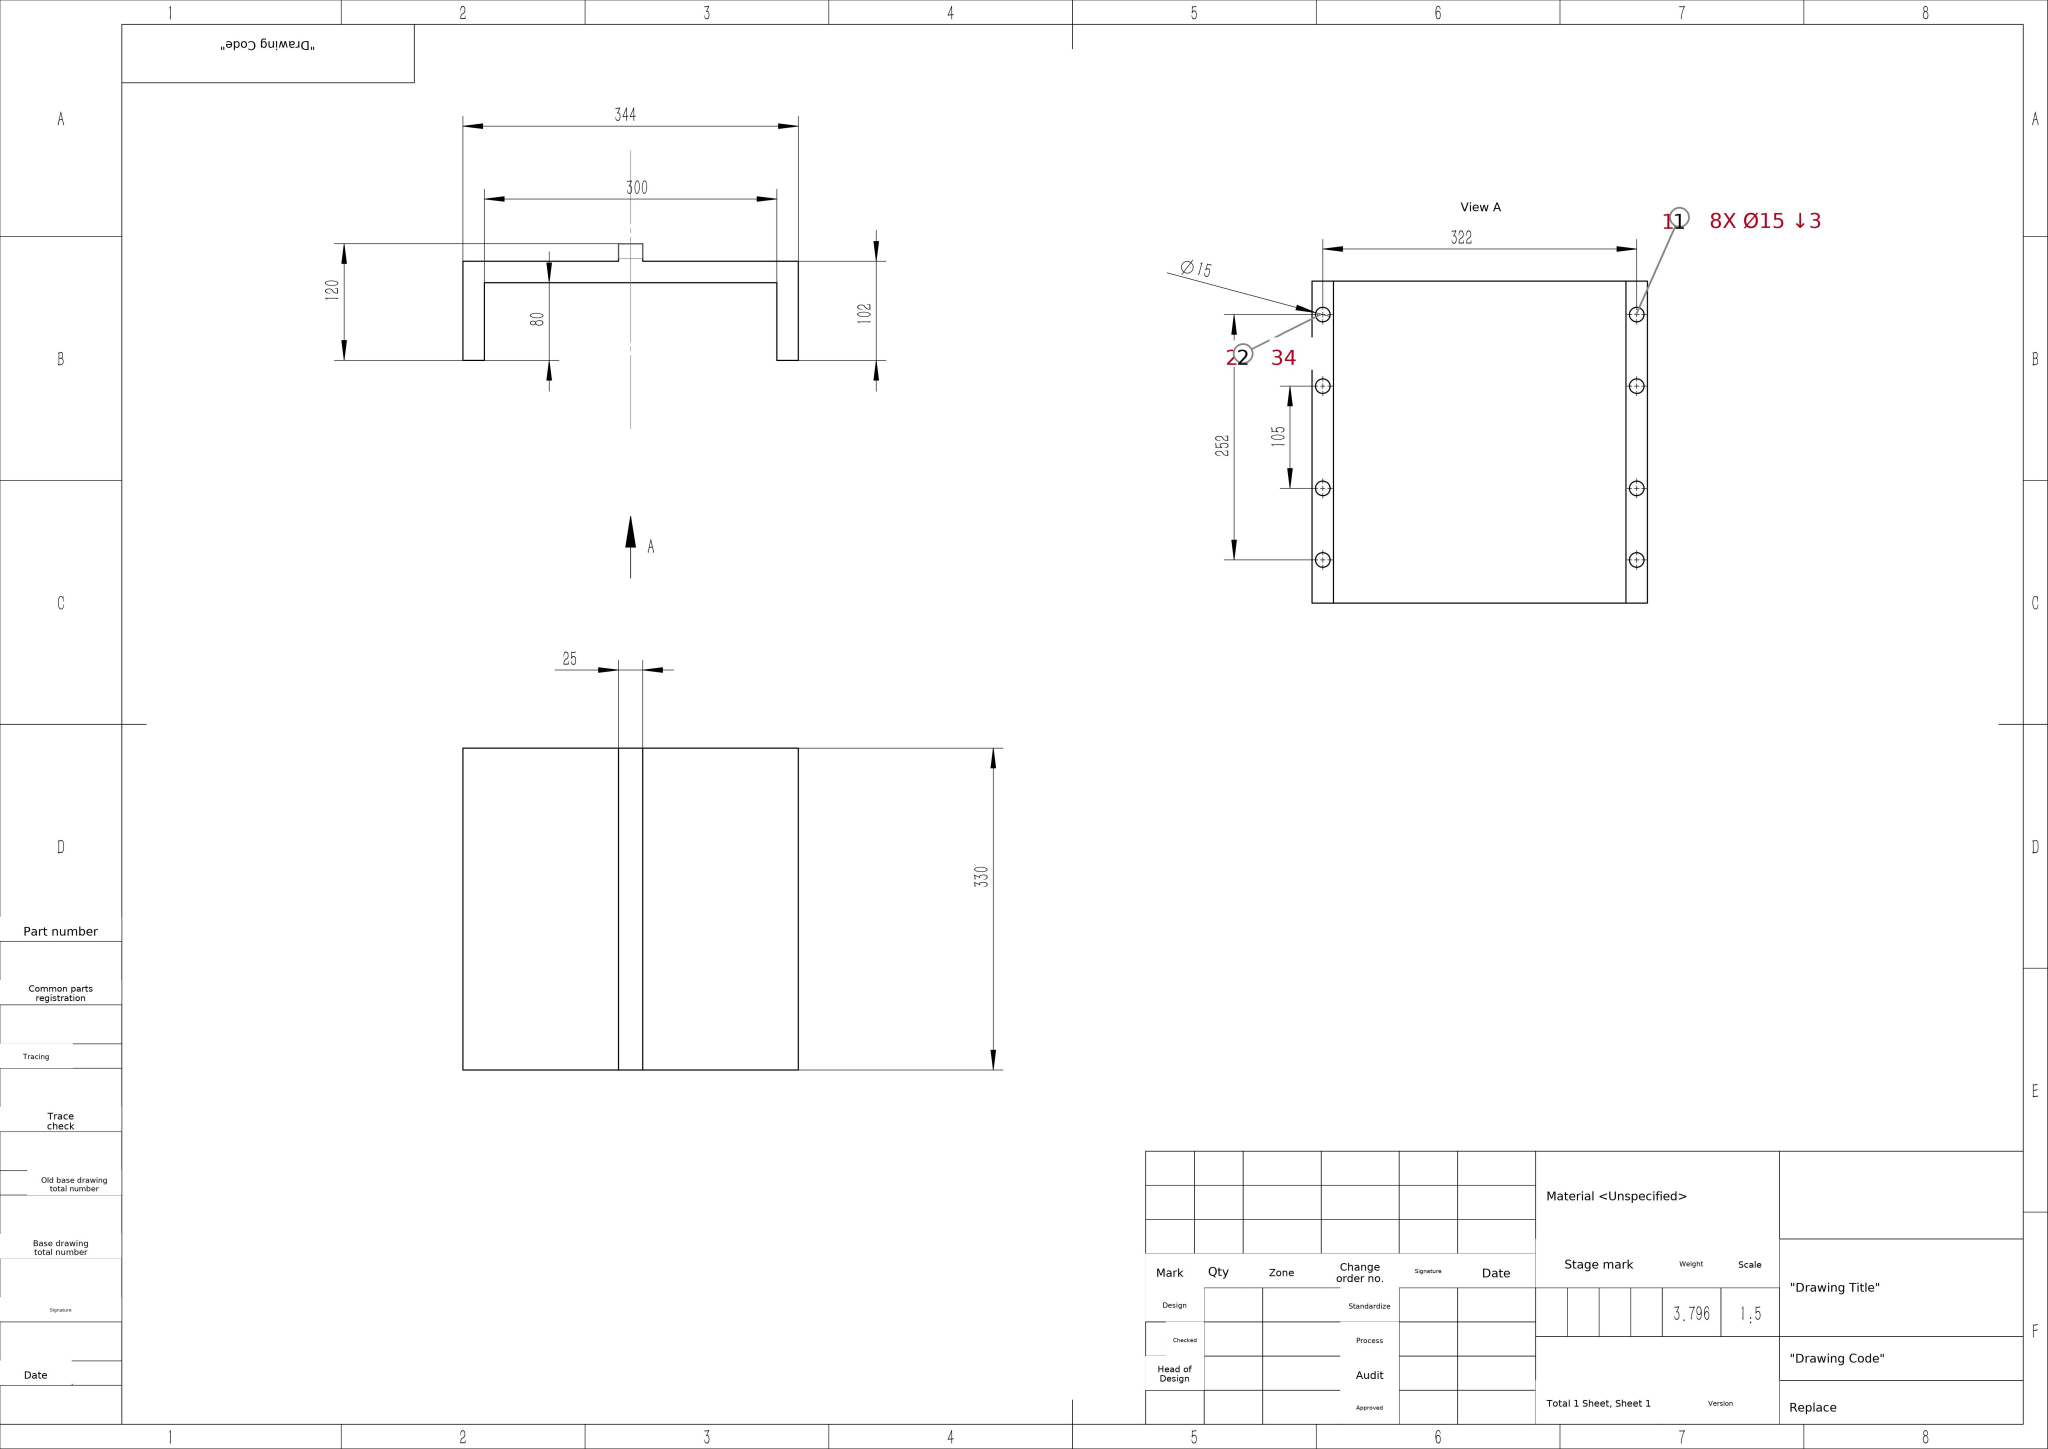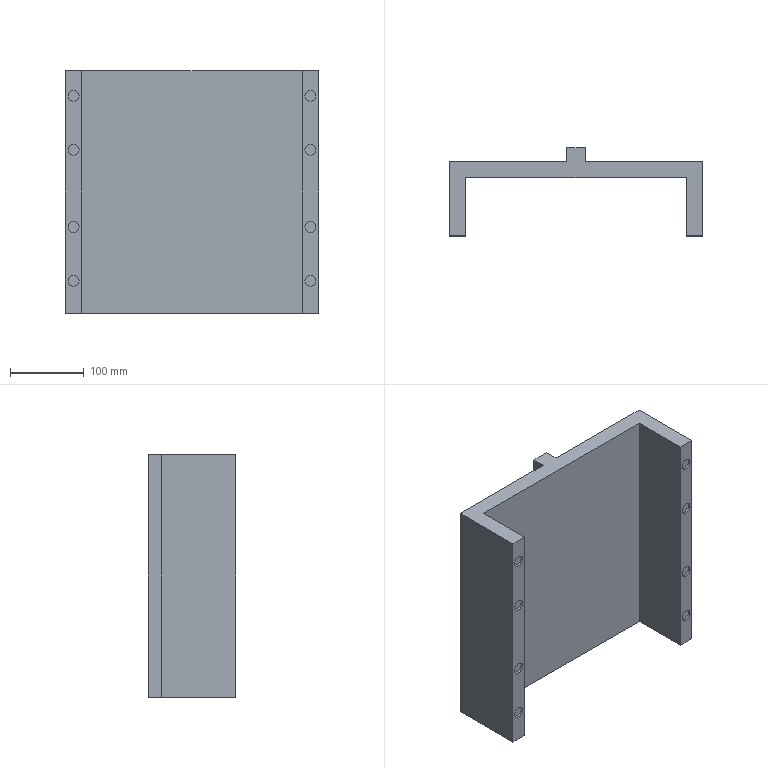Part | SolidWorks | mm | 1 solid | 38 faces | box 344 x 119.49 x 330 mm | volume 3795702 mm3 | plane 22 | cylinder 16 | commonest cylinder face diameters 15.01 x16
build123d program:
from build123d import *

# Parameters (mm, degrees)
SKETCH1_R           = 175
SKETCH1_R_2         = 135
BOSS_EXTRUDE1_DEPTH = 160
SKETCH2_W           = 25
SKETCH2_H           = 15
BOSS_EXTRUDE2_DEPTH = 160
SKETCH3_R           = 215
SKETCH3_R_2         = 135
BOSS_EXTRUDE3_DEPTH = 15
SKETCH4_R           = 7.525
CUT_EXTRUDE1_DEPTH  = 3
SKETCH6_W           = 350
SKETCH6_H           = 349.553
SKETCH6_W_2         = 300
SKETCH6_H_2         = 299.553
BOSS_EXTRUDE4_DEPTH = 145
SKETCH7_W           = 300
SKETCH7_H           = 299.553
CUT_EXTRUDE2_DEPTH  = 646
SKETCH8_W           = 430
SKETCH8_H           = 430
BOSS_EXTRUDE5_DEPTH = 15
SKETCH9_W           = 300
SKETCH9_H           = 299.553
CUT_EXTRUDE3_DEPTH  = 38
SKETCH11_R          = 7.525
CUT_EXTRUDE4_DEPTH  = 3
SKETCH12_W          = 457.43
SKETCH12_H          = 449.34
CUT_EXTRUDE7_DEPTH  = 145
SKETCH13_R          = 376.544
CUT_EXTRUDE8_DEPTH  = 176
SKETCH14_W          = 707.733
SKETCH14_H          = 268.113
CUT_EXTRUDE9_DEPTH  = 176
BOSS_EXTRUDE6_DEPTH = 185
SKETCH17_R          = 7.505
CUT_EXTRUDE10_DEPTH = 3.01


with BuildPart() as part:
    # Sketch1 → Boss-Extrude1 (new body)
    with BuildSketch(Plane.XY):
        Circle(SKETCH1_R)
        Circle(SKETCH1_R_2, mode=Mode.SUBTRACT)
    extrude(amount=BOSS_EXTRUDE1_DEPTH)

    # Sketch2 → Boss-Extrude2 (add)
    with BuildSketch(Plane(origin=(0, 0, 0), x_dir=(-1, 0, 0), z_dir=(0, 0, -1))):
        with Locations((0, 182.053)):
            Rectangle(SKETCH2_W, SKETCH2_H)
    extrude(amount=-BOSS_EXTRUDE2_DEPTH)

    # Sketch3 → Boss-Extrude3 (add)
    with BuildSketch(Plane(origin=(0, 0, 0), x_dir=(-1, 0, 0), z_dir=(0, 0, -1))):
        Circle(SKETCH3_R)
        with Locations(Location((0, 0, 0), (0, 0, 180))):
            Circle(SKETCH3_R_2, mode=Mode.SUBTRACT)
    extrude(amount=-BOSS_EXTRUDE3_DEPTH)

    # Sketch4 → Cut-Extrude1 (cut)
    with BuildSketch(Plane(origin=(0, 0, 0), x_dir=(-1, 0, 0), z_dir=(0, 0, -1))):
        with Locations((0, 170)):
            Circle(SKETCH4_R)
        with Locations((120.208, 120.208)):
            Circle(SKETCH4_R)
        with Locations((170, 0)):
            Circle(SKETCH4_R)
        with Locations((120.208, -120.208)):
            Circle(SKETCH4_R)
        with Locations((0, -170)):
            Circle(SKETCH4_R)
        with Locations((-120.208, -120.208)):
            Circle(SKETCH4_R)
        with Locations((-170, 0)):
            Circle(SKETCH4_R)
        with Locations((-120.208, 120.208)):
            Circle(SKETCH4_R)
    extrude(amount=-CUT_EXTRUDE1_DEPTH, mode=Mode.SUBTRACT)

    # Sketch6 → Boss-Extrude4 (add)
    with BuildSketch(Plane.XY.offset(160)):
        with Locations((0, -0.2235)):
            Rectangle(SKETCH6_W, SKETCH6_H)
        with Locations((0, -0.2235)):
            Rectangle(SKETCH6_W_2, SKETCH6_H_2, mode=Mode.SUBTRACT)
    extrude(amount=-BOSS_EXTRUDE4_DEPTH)

    # Sketch7 → Cut-Extrude2 (cut)
    with BuildSketch(Plane.XY.offset(160)):
        with Locations((0, -0.2235)):
            Rectangle(SKETCH7_W, SKETCH7_H)
    extrude(amount=-CUT_EXTRUDE2_DEPTH, mode=Mode.SUBTRACT)

    # Sketch8 → Boss-Extrude5 (add)
    with BuildSketch(Plane(origin=(0, 0, 0), x_dir=(-1, 0, 0), z_dir=(0, 0, -1))):
        Rectangle(SKETCH8_W, SKETCH8_H)
    extrude(amount=-BOSS_EXTRUDE5_DEPTH)

    # Sketch9 → Cut-Extrude3 (cut)
    with BuildSketch(Plane.XY.offset(15)):
        with Locations((0, -0.2235)):
            Rectangle(SKETCH9_W, SKETCH9_H)
    extrude(amount=-CUT_EXTRUDE3_DEPTH, mode=Mode.SUBTRACT)

    # Sketch11 → Cut-Extrude4 (cut)
    with BuildSketch(Plane(origin=(0, 0, 0), x_dir=(-1, 0, 0), z_dir=(0, 0, -1))):
        with Locations((-185.679, 182.277)):
            Circle(SKETCH11_R)
        with Locations((185.679, 182.277)):
            Circle(SKETCH11_R)
        with Locations((185.679, -182.277)):
            Circle(SKETCH11_R)
        with Locations((-185.679, -182.277)):
            Circle(SKETCH11_R)
        with Locations((-185.679, 0)):
            Circle(SKETCH11_R)
        with Locations((0, 182.277)):
            Circle(SKETCH11_R)
        with Locations((0, -182.277)):
            Circle(SKETCH11_R)
        with Locations((185.679, 0)):
            Circle(SKETCH11_R)
    extrude(amount=-CUT_EXTRUDE4_DEPTH, mode=Mode.SUBTRACT)

    # Sketch12 → Cut-Extrude7 (cut)
    with BuildSketch(Plane.XY.offset(160)):
        Rectangle(SKETCH12_W, SKETCH12_H)
        Polygon((172, -171.553), (-172, -171.553), (-172, 171.553), (-12.45, 171.553), (-12.45, 189.493), (12.45, 189.493), (12.45, 171.553), (172, 171.553), align=None, mode=Mode.SUBTRACT)
    extrude(amount=-CUT_EXTRUDE7_DEPTH, mode=Mode.SUBTRACT)

    # Sketch13 → Cut-Extrude8 (cut)
    with BuildSketch(Plane.XY.offset(15)):
        Circle(SKETCH13_R)
    extrude(amount=-CUT_EXTRUDE8_DEPTH, mode=Mode.SUBTRACT)

    # Sketch14 → Cut-Extrude9 (cut)
    with BuildSketch(Plane(origin=(0, 0, 15), x_dir=(-1, 0, 0), z_dir=(0, 0, -1))):
        with Locations((-3.434, -64.056)):
            Rectangle(SKETCH14_W, SKETCH14_H)
    extrude(amount=-CUT_EXTRUDE9_DEPTH, mode=Mode.SUBTRACT)

    # Sketch16 → Boss-Extrude6 (add)
    with BuildSketch(Plane(origin=(0, 0, 15), x_dir=(-1, 0, 0), z_dir=(0, 0, -1))):
        Polygon((-172, 171.553), (-172, 70), (-150, 70), (-150, 149.553), (150, 149.553), (150, 70), (172, 70), (172, 171.553), (12.45, 171.553), (12.45, 189.493), (-12.45, 189.493), (-12.45, 171.553), align=None)
    extrude(amount=BOSS_EXTRUDE6_DEPTH)

    # Sketch17 → Cut-Extrude10 (cut)
    with BuildSketch(Plane.XZ.offset(-70)):
        with Locations((-161, 125.752)):
            Circle(SKETCH17_R)
        with Locations((-161, 52.384)):
            Circle(SKETCH17_R)
        with Locations(Location((-161, -52.384, 0), (0, 0, 180))):
            Circle(SKETCH17_R)
        with Locations(Location((-161, -125.752, 0), (0, 0, 180))):
            Circle(SKETCH17_R)
        with Locations((161, -125.752)):
            Circle(SKETCH17_R)
        with Locations((161, -52.384)):
            Circle(SKETCH17_R)
        with Locations(Location((161, 52.384, 0), (0, 0, 180))):
            Circle(SKETCH17_R)
        with Locations(Location((161, 125.752, 0), (0, 0, 180))):
            Circle(SKETCH17_R)
    extrude(amount=-CUT_EXTRUDE10_DEPTH, mode=Mode.SUBTRACT)


solid = part.part